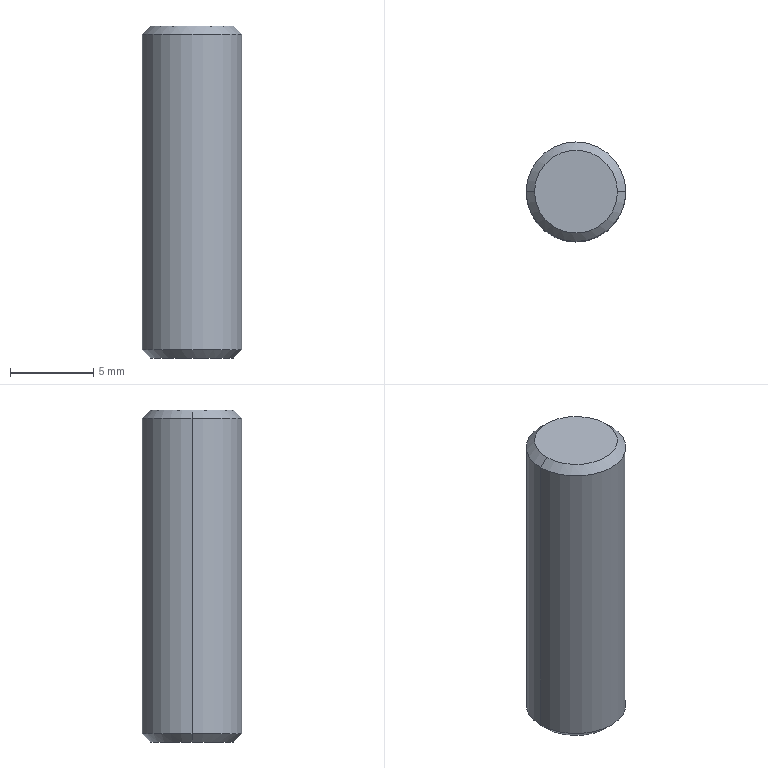Component | SolidWorks | BSH3-03-02RotatingPin-1 | 1 solid | 8 faces | box 6 x 6 x 20 mm | volume 561 mm3 | cone 4 | cylinder 2 | plane 2 | commonest cylinder face diameters 6 x2
build123d program:
from build123d import *

# Parameters (mm, degrees)
SKETCH1_R      = 3
EXTRUDE1_DEPTH = 20
CHAMFER1_SIZE  = 0.5


with BuildPart() as part:
    # Sketch1 → Extrude1 (new body)
    with BuildSketch(Plane.XY):
        Circle(SKETCH1_R)
    extrude(amount=EXTRUDE1_DEPTH)

    # Chamfer1
    chamfer1_edges = [part.edges().sort_by_distance(p)[0] for p in [
        (-3, 0, 0),
        (-3, 0, 20),
    ]]
    chamfer(chamfer1_edges, length=CHAMFER1_SIZE)


solid = part.part

# Placed as in the assembly
solid = solid.moved(Location((-108.621, -15.488, -11.439), (0, 0, 0)))
STEP:
#1=CARTESIAN_POINT('',(-4.178,-0.6098,0.337));
#2=VERTEX_POINT('',#1);
#3=CARTESIAN_POINT('',(-4.375,-0.6098,0.337));
#4=VERTEX_POINT('',#3);
#5=CARTESIAN_POINT('',(-4.276,-0.6098,0.337));
#6=DIRECTION('',(0.,0.,1.));
#7=DIRECTION('',(1.,0.,0.));
#8=AXIS2_PLACEMENT_3D('',#5,#6,#7);
#9=CIRCLE('',#8,0.09843);
#10=EDGE_CURVE('',#2,#4,#9,.T.);
#11=ORIENTED_EDGE('',*,*,#10,.F.);
#12=CARTESIAN_POINT('',(-4.158,-0.6098,0.3174));
#13=VERTEX_POINT('',#12);
#14=CARTESIAN_POINT('',(-4.178,-0.6098,0.337));
#15=DIRECTION('',(0.7071,0.,-0.7071));
#16=VECTOR('',#15,39.37);
#17=LINE('',#14,#16);
#18=EDGE_CURVE('',#2,#13,#17,.T.);
#19=ORIENTED_EDGE('',*,*,#18,.T.);
#20=CARTESIAN_POINT('',(-4.395,-0.6098,0.3174));
#21=VERTEX_POINT('',#20);
#22=CARTESIAN_POINT('',(-4.276,-0.6098,0.3174));
#23=DIRECTION('',(0.,0.,-1.));
#24=DIRECTION('',(1.,0.,0.));
#25=AXIS2_PLACEMENT_3D('',#22,#23,#24);
#26=CIRCLE('',#25,0.1181);
#27=EDGE_CURVE('',#21,#13,#26,.T.);
#28=ORIENTED_EDGE('',*,*,#27,.F.);
#29=CARTESIAN_POINT('',(-4.375,-0.6098,0.337));
#30=DIRECTION('',(-0.7071,0.,-0.7071));
#31=VECTOR('',#30,39.37);
#32=LINE('',#29,#31);
#33=EDGE_CURVE('',#4,#21,#32,.T.);
#34=ORIENTED_EDGE('',*,*,#33,.F.);
#35=EDGE_LOOP('',(#11,#19,#28,#34));
#36=FACE_OUTER_BOUND('',#35,.T.);
#37=CARTESIAN_POINT('',(-4.276,-0.6098,0.337));
#38=DIRECTION('',(0.,0.,-1.));
#39=DIRECTION('',(-1.,0.,0.));
#40=AXIS2_PLACEMENT_3D('',#37,#38,#39);
#41=CONICAL_SURFACE('',#40,0.09843,0.7854);
#42=ADVANCED_FACE('',(#36),#41,.T.);
#43=CARTESIAN_POINT('',(-4.375,-0.6098,-0.4504));
#44=VERTEX_POINT('',#43);
#45=CARTESIAN_POINT('',(-4.178,-0.6098,-0.4504));
#46=VERTEX_POINT('',#45);
#47=CARTESIAN_POINT('',(-4.276,-0.6098,-0.4504));
#48=DIRECTION('',(0.,0.,-1.));
#49=DIRECTION('',(1.,0.,0.));
#50=AXIS2_PLACEMENT_3D('',#47,#48,#49);
#51=CIRCLE('',#50,0.09843);
#52=EDGE_CURVE('',#44,#46,#51,.T.);
#53=ORIENTED_EDGE('',*,*,#52,.F.);
#54=CARTESIAN_POINT('',(-4.395,-0.6098,-0.4307));
#55=VERTEX_POINT('',#54);
#56=CARTESIAN_POINT('',(-4.395,-0.6098,-0.4307));
#57=DIRECTION('',(-0.7071,0.,0.7071));
#58=VECTOR('',#57,39.37);
#59=LINE('',#56,#58);
#60=EDGE_CURVE('',#44,#55,#59,.T.);
#61=ORIENTED_EDGE('',*,*,#60,.T.);
#62=CARTESIAN_POINT('',(-4.158,-0.6098,-0.4307));
#63=VERTEX_POINT('',#62);
#64=CARTESIAN_POINT('',(-4.276,-0.6098,-0.4307));
#65=DIRECTION('',(0.,0.,1.));
#66=DIRECTION('',(1.,0.,0.));
#67=AXIS2_PLACEMENT_3D('',#64,#65,#66);
#68=CIRCLE('',#67,0.1181);
#69=EDGE_CURVE('',#63,#55,#68,.T.);
#70=ORIENTED_EDGE('',*,*,#69,.F.);
#71=CARTESIAN_POINT('',(-4.158,-0.6098,-0.4307));
#72=DIRECTION('',(0.7071,0.,0.7071));
#73=VECTOR('',#72,39.37);
#74=LINE('',#71,#73);
#75=EDGE_CURVE('',#46,#63,#74,.T.);
#76=ORIENTED_EDGE('',*,*,#75,.F.);
#77=EDGE_LOOP('',(#53,#61,#70,#76));
#78=FACE_OUTER_BOUND('',#77,.T.);
#79=CARTESIAN_POINT('',(-4.276,-0.6098,-0.4307));
#80=DIRECTION('',(0.,0.,1.));
#81=DIRECTION('',(1.,0.,0.));
#82=AXIS2_PLACEMENT_3D('',#79,#80,#81);
#83=CONICAL_SURFACE('',#82,0.1181,0.7854);
#84=ADVANCED_FACE('',(#78),#83,.T.);
#85=ORIENTED_EDGE('',*,*,#27,.T.);
#86=CARTESIAN_POINT('',(-4.158,-0.6098,0.337));
#87=DIRECTION('',(0.,0.,-1.));
#88=VECTOR('',#87,39.37);
#89=LINE('',#86,#88);
#90=EDGE_CURVE('',#13,#63,#89,.T.);
#91=ORIENTED_EDGE('',*,*,#90,.T.);
#92=ORIENTED_EDGE('',*,*,#69,.T.);
#93=CARTESIAN_POINT('',(-4.395,-0.6098,0.337));
#94=DIRECTION('',(0.,0.,-1.));
#95=VECTOR('',#94,39.37);
#96=LINE('',#93,#95);
#97=EDGE_CURVE('',#21,#55,#96,.T.);
#98=ORIENTED_EDGE('',*,*,#97,.F.);
#99=EDGE_LOOP('',(#85,#91,#92,#98));
#100=FACE_OUTER_BOUND('',#99,.T.);
#101=CARTESIAN_POINT('',(-4.276,-0.6098,0.337));
#102=DIRECTION('',(0.,0.,-1.));
#103=DIRECTION('',(-1.,0.,0.));
#104=AXIS2_PLACEMENT_3D('',#101,#102,#103);
#105=CYLINDRICAL_SURFACE('',#104,0.1181);
#106=ADVANCED_FACE('',(#100),#105,.T.);
#107=ORIENTED_EDGE('',*,*,#90,.F.);
#108=CARTESIAN_POINT('',(-4.276,-0.6098,0.3174));
#109=DIRECTION('',(0.,0.,-1.));
#110=DIRECTION('',(1.,0.,0.));
#111=AXIS2_PLACEMENT_3D('',#108,#109,#110);
#112=CIRCLE('',#111,0.1181);
#113=EDGE_CURVE('',#13,#21,#112,.T.);
#114=ORIENTED_EDGE('',*,*,#113,.T.);
#115=ORIENTED_EDGE('',*,*,#97,.T.);
#116=CARTESIAN_POINT('',(-4.276,-0.6098,-0.4307));
#117=DIRECTION('',(0.,0.,1.));
#118=DIRECTION('',(1.,0.,0.));
#119=AXIS2_PLACEMENT_3D('',#116,#117,#118);
#120=CIRCLE('',#119,0.1181);
#121=EDGE_CURVE('',#55,#63,#120,.T.);
#122=ORIENTED_EDGE('',*,*,#121,.T.);
#123=EDGE_LOOP('',(#107,#114,#115,#122));
#124=FACE_OUTER_BOUND('',#123,.T.);
#125=CARTESIAN_POINT('',(-4.276,-0.6098,0.337));
#126=DIRECTION('',(0.,0.,-1.));
#127=DIRECTION('',(-1.,0.,0.));
#128=AXIS2_PLACEMENT_3D('',#125,#126,#127);
#129=CYLINDRICAL_SURFACE('',#128,0.1181);
#130=ADVANCED_FACE('',(#124),#129,.T.);
#131=CARTESIAN_POINT('',(-4.276,-0.6098,0.337));
#132=DIRECTION('',(0.,0.,1.));
#133=DIRECTION('',(1.,0.,0.));
#134=AXIS2_PLACEMENT_3D('',#131,#132,#133);
#135=CIRCLE('',#134,0.09843);
#136=EDGE_CURVE('',#4,#2,#135,.T.);
#137=ORIENTED_EDGE('',*,*,#136,.T.);
#138=ORIENTED_EDGE('',*,*,#10,.T.);
#139=EDGE_LOOP('',(#137,#138));
#140=FACE_OUTER_BOUND('',#139,.T.);
#141=CARTESIAN_POINT('',(-4.276,-0.6098,0.337));
#142=DIRECTION('',(0.,0.,1.));
#143=DIRECTION('',(1.,0.,0.));
#144=AXIS2_PLACEMENT_3D('',#141,#142,#143);
#145=PLANE('',#144);
#146=ADVANCED_FACE('',(#140),#145,.T.);
#147=CARTESIAN_POINT('',(-4.276,-0.6098,-0.4504));
#148=DIRECTION('',(0.,0.,-1.));
#149=DIRECTION('',(1.,0.,0.));
#150=AXIS2_PLACEMENT_3D('',#147,#148,#149);
#151=CIRCLE('',#150,0.09843);
#152=EDGE_CURVE('',#46,#44,#151,.T.);
#153=ORIENTED_EDGE('',*,*,#152,.T.);
#154=ORIENTED_EDGE('',*,*,#52,.T.);
#155=EDGE_LOOP('',(#153,#154));
#156=FACE_OUTER_BOUND('',#155,.T.);
#157=CARTESIAN_POINT('',(-4.276,-0.6098,-0.4504));
#158=DIRECTION('',(0.,0.,1.));
#159=DIRECTION('',(1.,0.,0.));
#160=AXIS2_PLACEMENT_3D('',#157,#158,#159);
#161=PLANE('',#160);
#162=ADVANCED_FACE('',(#156),#161,.F.);
#163=ORIENTED_EDGE('',*,*,#60,.F.);
#164=ORIENTED_EDGE('',*,*,#152,.F.);
#165=ORIENTED_EDGE('',*,*,#75,.T.);
#166=ORIENTED_EDGE('',*,*,#121,.F.);
#167=EDGE_LOOP('',(#163,#164,#165,#166));
#168=FACE_OUTER_BOUND('',#167,.T.);
#169=CARTESIAN_POINT('',(-4.276,-0.6098,-0.4307));
#170=DIRECTION('',(0.,0.,1.));
#171=DIRECTION('',(1.,0.,0.));
#172=AXIS2_PLACEMENT_3D('',#169,#170,#171);
#173=CONICAL_SURFACE('',#172,0.1181,0.7854);
#174=ADVANCED_FACE('',(#168),#173,.T.);
#175=ORIENTED_EDGE('',*,*,#18,.F.);
#176=ORIENTED_EDGE('',*,*,#136,.F.);
#177=ORIENTED_EDGE('',*,*,#33,.T.);
#178=ORIENTED_EDGE('',*,*,#113,.F.);
#179=EDGE_LOOP('',(#175,#176,#177,#178));
#180=FACE_OUTER_BOUND('',#179,.T.);
#181=CARTESIAN_POINT('',(-4.276,-0.6098,0.337));
#182=DIRECTION('',(0.,0.,-1.));
#183=DIRECTION('',(-1.,0.,0.));
#184=AXIS2_PLACEMENT_3D('',#181,#182,#183);
#185=CONICAL_SURFACE('',#184,0.09843,0.7854);
#186=ADVANCED_FACE('',(#180),#185,.T.);
#187=CLOSED_SHELL('',(#42,#84,#106,#130,#146,#162,#174,#186));
#188=MANIFOLD_SOLID_BREP('',#187);
#189=CARTESIAN_POINT('',(0.,0.,0.));
#190=DIRECTION('',(0.,0.,1.));
#191=DIRECTION('',(1.,0.,0.));
#192=AXIS2_PLACEMENT_3D('',#189,#190,#191);
#193=(LENGTH_UNIT()NAMED_UNIT(*)SI_UNIT($,.METRE.));
#194=LENGTH_MEASURE_WITH_UNIT(LENGTH_MEASURE(0.0254),#193);
#195=DIMENSIONAL_EXPONENTS(1.,0.,0.,0.,0.,0.,0.);
#196=(CONVERSION_BASED_UNIT('',#194)LENGTH_UNIT()NAMED_UNIT(#195));
#197=UNCERTAINTY_MEASURE_WITH_UNIT(LENGTH_MEASURE(0.00001),#196,'','');
#198=(NAMED_UNIT(*)PLANE_ANGLE_UNIT()SI_UNIT($,.RADIAN.));
#199=(NAMED_UNIT(*)SI_UNIT($,.STERADIAN.)SOLID_ANGLE_UNIT());
#200=(GEOMETRIC_REPRESENTATION_CONTEXT(3)GLOBAL_UNCERTAINTY_ASSIGNED_CONTEXT((#197))GLOBAL_UNIT_ASSIGNED_CONTEXT((#196,#198,#199))REPRESENTATION_CONTEXT('',''));
#201=ADVANCED_BREP_SHAPE_REPRESENTATION('',(#188,#192),#200);
#202=COLOUR_RGB('',0.7922,0.8196,0.9333);
#203=FILL_AREA_STYLE_COLOUR('',#202);
#204=FILL_AREA_STYLE('',(#203));
#205=SURFACE_STYLE_FILL_AREA(#204);
#206=SURFACE_SIDE_STYLE('',(#205));
#207=SURFACE_STYLE_USAGE(.BOTH.,#206);
#208=PRESENTATION_STYLE_ASSIGNMENT((#207));
#209=STYLED_ITEM('',(#208),#188);
#210=(LENGTH_UNIT()NAMED_UNIT(*)SI_UNIT($,.METRE.));
#211=LENGTH_MEASURE_WITH_UNIT(LENGTH_MEASURE(0.0254),#210);
#212=DIMENSIONAL_EXPONENTS(1.,0.,0.,0.,0.,0.,0.);
#213=(CONVERSION_BASED_UNIT('',#211)LENGTH_UNIT()NAMED_UNIT(#212));
#214=UNCERTAINTY_MEASURE_WITH_UNIT(LENGTH_MEASURE(0.00001),#213,'','');
#215=(NAMED_UNIT(*)PLANE_ANGLE_UNIT()SI_UNIT($,.RADIAN.));
#216=(NAMED_UNIT(*)SI_UNIT($,.STERADIAN.)SOLID_ANGLE_UNIT());
#217=(GEOMETRIC_REPRESENTATION_CONTEXT(3)GLOBAL_UNCERTAINTY_ASSIGNED_CONTEXT((#214))GLOBAL_UNIT_ASSIGNED_CONTEXT((#213,#215,#216))REPRESENTATION_CONTEXT('',''));
#218=MECHANICAL_DESIGN_GEOMETRIC_PRESENTATION_REPRESENTATION('',(#209),#217);
#219=PRESENTATION_LAYER_ASSIGNMENT('','',(#209));